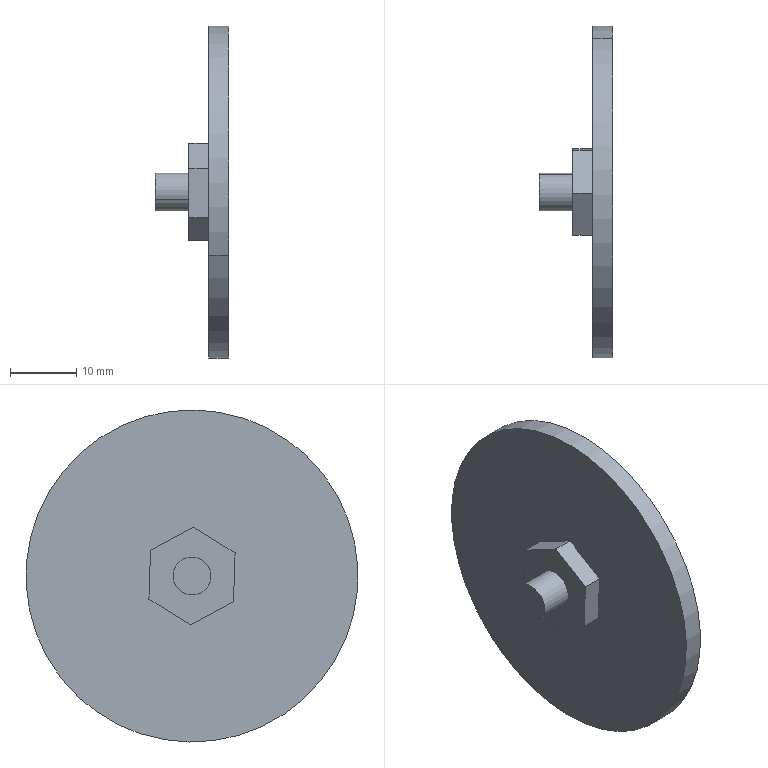Component | SolidWorks | RetainingRing,Gasket,Bolt-4 | 1 solid | 14 faces | box 11 x 50 x 50 mm | volume 6440 mm3 | plane 10 | cylinder 4 | commonest cylinder face diameters 5.711 x2 50 x2
STEP:
#1=CARTESIAN_POINT('',(3.485,0.7067,-4.288));
#2=VERTEX_POINT('',#1);
#3=CARTESIAN_POINT('',(3.485,0.4989,-4.374));
#4=VERTEX_POINT('',#3);
#5=CARTESIAN_POINT('',(3.485,0.6028,-4.331));
#6=DIRECTION('',(-1.,0.,0.));
#7=DIRECTION('',(0.,0.9242,0.3818));
#8=AXIS2_PLACEMENT_3D('',#5,#6,#7);
#9=CIRCLE('',#8,0.1124);
#10=EDGE_CURVE('',#2,#4,#9,.T.);
#11=ORIENTED_EDGE('',*,*,#10,.F.);
#12=CARTESIAN_POINT('',(3.682,0.7067,-4.288));
#13=VERTEX_POINT('',#12);
#14=CARTESIAN_POINT('',(3.485,0.7067,-4.288));
#15=DIRECTION('',(1.,0.,0.));
#16=VECTOR('',#15,39.37);
#17=LINE('',#14,#16);
#18=EDGE_CURVE('',#2,#13,#17,.T.);
#19=ORIENTED_EDGE('',*,*,#18,.T.);
#20=CARTESIAN_POINT('',(3.682,0.4989,-4.374));
#21=VERTEX_POINT('',#20);
#22=CARTESIAN_POINT('',(3.682,0.6028,-4.331));
#23=DIRECTION('',(-1.,0.,0.));
#24=DIRECTION('',(0.,0.9242,0.3818));
#25=AXIS2_PLACEMENT_3D('',#22,#23,#24);
#26=CIRCLE('',#25,0.1124);
#27=EDGE_CURVE('',#13,#21,#26,.T.);
#28=ORIENTED_EDGE('',*,*,#27,.T.);
#29=CARTESIAN_POINT('',(3.485,0.4989,-4.374));
#30=DIRECTION('',(1.,0.,0.));
#31=VECTOR('',#30,39.37);
#32=LINE('',#29,#31);
#33=EDGE_CURVE('',#4,#21,#32,.T.);
#34=ORIENTED_EDGE('',*,*,#33,.F.);
#35=EDGE_LOOP('',(#11,#19,#28,#34));
#36=FACE_OUTER_BOUND('',#35,.T.);
#37=CARTESIAN_POINT('',(3.485,0.6028,-4.331));
#38=DIRECTION('',(1.,0.,0.));
#39=DIRECTION('',(0.,-0.9242,-0.3818));
#40=AXIS2_PLACEMENT_3D('',#37,#38,#39);
#41=CYLINDRICAL_SURFACE('',#40,0.1124);
#42=ADVANCED_FACE('',(#36),#41,.T.);
#43=CARTESIAN_POINT('',(3.8,1.512,-3.955));
#44=VERTEX_POINT('',#43);
#45=CARTESIAN_POINT('',(3.8,-0.3069,-4.707));
#46=VERTEX_POINT('',#45);
#47=CARTESIAN_POINT('',(3.8,0.6028,-4.331));
#48=DIRECTION('',(-1.,0.,0.));
#49=DIRECTION('',(0.,0.9242,0.3818));
#50=AXIS2_PLACEMENT_3D('',#47,#48,#49);
#51=CIRCLE('',#50,0.9843);
#52=EDGE_CURVE('',#44,#46,#51,.T.);
#53=ORIENTED_EDGE('',*,*,#52,.F.);
#54=CARTESIAN_POINT('',(3.918,1.512,-3.955));
#55=VERTEX_POINT('',#54);
#56=CARTESIAN_POINT('',(3.8,1.512,-3.955));
#57=DIRECTION('',(1.,0.,0.));
#58=VECTOR('',#57,39.37);
#59=LINE('',#56,#58);
#60=EDGE_CURVE('',#44,#55,#59,.T.);
#61=ORIENTED_EDGE('',*,*,#60,.T.);
#62=CARTESIAN_POINT('',(3.918,-0.3069,-4.707));
#63=VERTEX_POINT('',#62);
#64=CARTESIAN_POINT('',(3.918,0.6028,-4.331));
#65=DIRECTION('',(-1.,0.,0.));
#66=DIRECTION('',(0.,0.9242,0.3818));
#67=AXIS2_PLACEMENT_3D('',#64,#65,#66);
#68=CIRCLE('',#67,0.9843);
#69=EDGE_CURVE('',#55,#63,#68,.T.);
#70=ORIENTED_EDGE('',*,*,#69,.T.);
#71=CARTESIAN_POINT('',(3.8,-0.3069,-4.707));
#72=DIRECTION('',(1.,0.,0.));
#73=VECTOR('',#72,39.37);
#74=LINE('',#71,#73);
#75=EDGE_CURVE('',#46,#63,#74,.T.);
#76=ORIENTED_EDGE('',*,*,#75,.F.);
#77=EDGE_LOOP('',(#53,#61,#70,#76));
#78=FACE_OUTER_BOUND('',#77,.T.);
#79=CARTESIAN_POINT('',(3.8,0.6028,-4.331));
#80=DIRECTION('',(1.,0.,0.));
#81=DIRECTION('',(0.,-0.9242,-0.3818));
#82=AXIS2_PLACEMENT_3D('',#79,#80,#81);
#83=CYLINDRICAL_SURFACE('',#82,0.9843);
#84=ADVANCED_FACE('',(#78),#83,.T.);
#85=CARTESIAN_POINT('',(3.682,0.3567,-4.483));
#86=VERTEX_POINT('',#85);
#87=CARTESIAN_POINT('',(3.682,0.3474,-4.194));
#88=VERTEX_POINT('',#87);
#89=CARTESIAN_POINT('',(3.682,0.3567,-4.483));
#90=DIRECTION('',(0.,-0.03186,0.9995));
#91=VECTOR('',#90,39.37);
#92=LINE('',#89,#91);
#93=EDGE_CURVE('',#86,#88,#92,.T.);
#94=ORIENTED_EDGE('',*,*,#93,.T.);
#95=CARTESIAN_POINT('',(3.682,0.5935,-4.041));
#96=VERTEX_POINT('',#95);
#97=CARTESIAN_POINT('',(3.682,0.3474,-4.194));
#98=DIRECTION('',(0.,0.8497,0.5273));
#99=VECTOR('',#98,39.37);
#100=LINE('',#97,#99);
#101=EDGE_CURVE('',#88,#96,#100,.T.);
#102=ORIENTED_EDGE('',*,*,#101,.T.);
#103=CARTESIAN_POINT('',(3.682,0.8489,-4.178));
#104=VERTEX_POINT('',#103);
#105=CARTESIAN_POINT('',(3.682,0.5935,-4.041));
#106=DIRECTION('',(0.,0.8815,-0.4722));
#107=VECTOR('',#106,39.37);
#108=LINE('',#105,#107);
#109=EDGE_CURVE('',#96,#104,#108,.T.);
#110=ORIENTED_EDGE('',*,*,#109,.T.);
#111=CARTESIAN_POINT('',(3.682,0.8581,-4.467));
#112=VERTEX_POINT('',#111);
#113=CARTESIAN_POINT('',(3.682,0.8489,-4.178));
#114=DIRECTION('',(0.,0.03186,-0.9995));
#115=VECTOR('',#114,39.37);
#116=LINE('',#113,#115);
#117=EDGE_CURVE('',#104,#112,#116,.T.);
#118=ORIENTED_EDGE('',*,*,#117,.T.);
#119=CARTESIAN_POINT('',(3.682,0.612,-4.62));
#120=VERTEX_POINT('',#119);
#121=CARTESIAN_POINT('',(3.682,0.8581,-4.467));
#122=DIRECTION('',(0.,-0.8497,-0.5273));
#123=VECTOR('',#122,39.37);
#124=LINE('',#121,#123);
#125=EDGE_CURVE('',#112,#120,#124,.T.);
#126=ORIENTED_EDGE('',*,*,#125,.T.);
#127=CARTESIAN_POINT('',(3.682,0.612,-4.62));
#128=DIRECTION('',(0.,-0.8815,0.4722));
#129=VECTOR('',#128,39.37);
#130=LINE('',#127,#129);
#131=EDGE_CURVE('',#120,#86,#130,.T.);
#132=ORIENTED_EDGE('',*,*,#131,.T.);
#133=EDGE_LOOP('',(#94,#102,#110,#118,#126,#132));
#134=FACE_OUTER_BOUND('',#133,.T.);
#135=CARTESIAN_POINT('',(3.682,0.6028,-4.331));
#136=DIRECTION('',(-1.,0.,0.));
#137=DIRECTION('',(0.,0.9242,0.3818));
#138=AXIS2_PLACEMENT_3D('',#135,#136,#137);
#139=CIRCLE('',#138,0.1124);
#140=EDGE_CURVE('',#21,#13,#139,.T.);
#141=ORIENTED_EDGE('',*,*,#140,.F.);
#142=ORIENTED_EDGE('',*,*,#27,.F.);
#143=EDGE_LOOP('',(#141,#142));
#144=FACE_BOUND('',#143,.T.);
#145=CARTESIAN_POINT('',(3.682,0.6028,-4.331));
#146=DIRECTION('',(-1.,0.,0.));
#147=DIRECTION('',(0.,0.9242,0.3818));
#148=AXIS2_PLACEMENT_3D('',#145,#146,#147);
#149=PLANE('',#148);
#150=ADVANCED_FACE('',(#134,#144),#149,.T.);
#151=CARTESIAN_POINT('',(3.8,0.6028,-4.331));
#152=DIRECTION('',(-1.,0.,0.));
#153=DIRECTION('',(0.,0.9242,0.3818));
#154=AXIS2_PLACEMENT_3D('',#151,#152,#153);
#155=CIRCLE('',#154,0.9843);
#156=EDGE_CURVE('',#46,#44,#155,.T.);
#157=ORIENTED_EDGE('',*,*,#156,.T.);
#158=ORIENTED_EDGE('',*,*,#52,.T.);
#159=EDGE_LOOP('',(#157,#158));
#160=FACE_OUTER_BOUND('',#159,.T.);
#161=CARTESIAN_POINT('',(3.8,0.3474,-4.194));
#162=VERTEX_POINT('',#161);
#163=CARTESIAN_POINT('',(3.8,0.5935,-4.041));
#164=VERTEX_POINT('',#163);
#165=CARTESIAN_POINT('',(3.8,0.3474,-4.194));
#166=DIRECTION('',(0.,0.8497,0.5273));
#167=VECTOR('',#166,39.37);
#168=LINE('',#165,#167);
#169=EDGE_CURVE('',#162,#164,#168,.T.);
#170=ORIENTED_EDGE('',*,*,#169,.F.);
#171=CARTESIAN_POINT('',(3.8,0.3567,-4.483));
#172=VERTEX_POINT('',#171);
#173=CARTESIAN_POINT('',(3.8,0.3567,-4.483));
#174=DIRECTION('',(0.,-0.03186,0.9995));
#175=VECTOR('',#174,39.37);
#176=LINE('',#173,#175);
#177=EDGE_CURVE('',#172,#162,#176,.T.);
#178=ORIENTED_EDGE('',*,*,#177,.F.);
#179=CARTESIAN_POINT('',(3.8,0.612,-4.62));
#180=VERTEX_POINT('',#179);
#181=CARTESIAN_POINT('',(3.8,0.612,-4.62));
#182=DIRECTION('',(0.,-0.8815,0.4722));
#183=VECTOR('',#182,39.37);
#184=LINE('',#181,#183);
#185=EDGE_CURVE('',#180,#172,#184,.T.);
#186=ORIENTED_EDGE('',*,*,#185,.F.);
#187=CARTESIAN_POINT('',(3.8,0.8581,-4.467));
#188=VERTEX_POINT('',#187);
#189=CARTESIAN_POINT('',(3.8,0.8581,-4.467));
#190=DIRECTION('',(0.,-0.8497,-0.5273));
#191=VECTOR('',#190,39.37);
#192=LINE('',#189,#191);
#193=EDGE_CURVE('',#188,#180,#192,.T.);
#194=ORIENTED_EDGE('',*,*,#193,.F.);
#195=CARTESIAN_POINT('',(3.8,0.8489,-4.178));
#196=VERTEX_POINT('',#195);
#197=CARTESIAN_POINT('',(3.8,0.8489,-4.178));
#198=DIRECTION('',(0.,0.03186,-0.9995));
#199=VECTOR('',#198,39.37);
#200=LINE('',#197,#199);
#201=EDGE_CURVE('',#196,#188,#200,.T.);
#202=ORIENTED_EDGE('',*,*,#201,.F.);
#203=CARTESIAN_POINT('',(3.8,0.5935,-4.041));
#204=DIRECTION('',(0.,0.8815,-0.4722));
#205=VECTOR('',#204,39.37);
#206=LINE('',#203,#205);
#207=EDGE_CURVE('',#164,#196,#206,.T.);
#208=ORIENTED_EDGE('',*,*,#207,.F.);
#209=EDGE_LOOP('',(#170,#178,#186,#194,#202,#208));
#210=FACE_BOUND('',#209,.T.);
#211=CARTESIAN_POINT('',(3.8,0.6028,-4.331));
#212=DIRECTION('',(-1.,0.,0.));
#213=DIRECTION('',(0.,0.9242,0.3818));
#214=AXIS2_PLACEMENT_3D('',#211,#212,#213);
#215=PLANE('',#214);
#216=ADVANCED_FACE('',(#160,#210),#215,.T.);
#217=ORIENTED_EDGE('',*,*,#60,.F.);
#218=ORIENTED_EDGE('',*,*,#156,.F.);
#219=ORIENTED_EDGE('',*,*,#75,.T.);
#220=CARTESIAN_POINT('',(3.918,0.6028,-4.331));
#221=DIRECTION('',(-1.,0.,0.));
#222=DIRECTION('',(0.,0.9242,0.3818));
#223=AXIS2_PLACEMENT_3D('',#220,#221,#222);
#224=CIRCLE('',#223,0.9843);
#225=EDGE_CURVE('',#63,#55,#224,.T.);
#226=ORIENTED_EDGE('',*,*,#225,.T.);
#227=EDGE_LOOP('',(#217,#218,#219,#226));
#228=FACE_OUTER_BOUND('',#227,.T.);
#229=CARTESIAN_POINT('',(3.8,0.6028,-4.331));
#230=DIRECTION('',(1.,0.,0.));
#231=DIRECTION('',(0.,-0.9242,-0.3818));
#232=AXIS2_PLACEMENT_3D('',#229,#230,#231);
#233=CYLINDRICAL_SURFACE('',#232,0.9843);
#234=ADVANCED_FACE('',(#228),#233,.T.);
#235=ORIENTED_EDGE('',*,*,#225,.F.);
#236=ORIENTED_EDGE('',*,*,#69,.F.);
#237=EDGE_LOOP('',(#235,#236));
#238=FACE_OUTER_BOUND('',#237,.T.);
#239=CARTESIAN_POINT('',(3.918,0.6028,-4.331));
#240=DIRECTION('',(-1.,0.,0.));
#241=DIRECTION('',(0.,0.9242,0.3818));
#242=AXIS2_PLACEMENT_3D('',#239,#240,#241);
#243=PLANE('',#242);
#244=ADVANCED_FACE('',(#238),#243,.F.);
#245=ORIENTED_EDGE('',*,*,#177,.T.);
#246=CARTESIAN_POINT('',(3.682,0.3474,-4.194));
#247=DIRECTION('',(1.,0.,0.));
#248=VECTOR('',#247,39.37);
#249=LINE('',#246,#248);
#250=EDGE_CURVE('',#88,#162,#249,.T.);
#251=ORIENTED_EDGE('',*,*,#250,.F.);
#252=ORIENTED_EDGE('',*,*,#93,.F.);
#253=CARTESIAN_POINT('',(3.682,0.3567,-4.483));
#254=DIRECTION('',(1.,0.,0.));
#255=VECTOR('',#254,39.37);
#256=LINE('',#253,#255);
#257=EDGE_CURVE('',#86,#172,#256,.T.);
#258=ORIENTED_EDGE('',*,*,#257,.T.);
#259=EDGE_LOOP('',(#245,#251,#252,#258));
#260=FACE_OUTER_BOUND('',#259,.T.);
#261=CARTESIAN_POINT('',(3.682,0.3567,-4.483));
#262=DIRECTION('',(0.,0.9995,0.03186));
#263=DIRECTION('',(0.,0.03186,-0.9995));
#264=AXIS2_PLACEMENT_3D('',#261,#262,#263);
#265=PLANE('',#264);
#266=ADVANCED_FACE('',(#260),#265,.F.);
#267=ORIENTED_EDGE('',*,*,#169,.T.);
#268=CARTESIAN_POINT('',(3.682,0.5935,-4.041));
#269=DIRECTION('',(1.,0.,0.));
#270=VECTOR('',#269,39.37);
#271=LINE('',#268,#270);
#272=EDGE_CURVE('',#96,#164,#271,.T.);
#273=ORIENTED_EDGE('',*,*,#272,.F.);
#274=ORIENTED_EDGE('',*,*,#101,.F.);
#275=ORIENTED_EDGE('',*,*,#250,.T.);
#276=EDGE_LOOP('',(#267,#273,#274,#275));
#277=FACE_OUTER_BOUND('',#276,.T.);
#278=CARTESIAN_POINT('',(3.682,0.3474,-4.194));
#279=DIRECTION('',(0.,0.5273,-0.8497));
#280=DIRECTION('',(0.,-0.8497,-0.5273));
#281=AXIS2_PLACEMENT_3D('',#278,#279,#280);
#282=PLANE('',#281);
#283=ADVANCED_FACE('',(#277),#282,.F.);
#284=ORIENTED_EDGE('',*,*,#207,.T.);
#285=CARTESIAN_POINT('',(3.682,0.8489,-4.178));
#286=DIRECTION('',(1.,0.,0.));
#287=VECTOR('',#286,39.37);
#288=LINE('',#285,#287);
#289=EDGE_CURVE('',#104,#196,#288,.T.);
#290=ORIENTED_EDGE('',*,*,#289,.F.);
#291=ORIENTED_EDGE('',*,*,#109,.F.);
#292=ORIENTED_EDGE('',*,*,#272,.T.);
#293=EDGE_LOOP('',(#284,#290,#291,#292));
#294=FACE_OUTER_BOUND('',#293,.T.);
#295=CARTESIAN_POINT('',(3.682,0.5935,-4.041));
#296=DIRECTION('',(0.,-0.4722,-0.8815));
#297=DIRECTION('',(0.,-0.8815,0.4722));
#298=AXIS2_PLACEMENT_3D('',#295,#296,#297);
#299=PLANE('',#298);
#300=ADVANCED_FACE('',(#294),#299,.F.);
#301=ORIENTED_EDGE('',*,*,#201,.T.);
#302=CARTESIAN_POINT('',(3.682,0.8581,-4.467));
#303=DIRECTION('',(1.,0.,0.));
#304=VECTOR('',#303,39.37);
#305=LINE('',#302,#304);
#306=EDGE_CURVE('',#112,#188,#305,.T.);
#307=ORIENTED_EDGE('',*,*,#306,.F.);
#308=ORIENTED_EDGE('',*,*,#117,.F.);
#309=ORIENTED_EDGE('',*,*,#289,.T.);
#310=EDGE_LOOP('',(#301,#307,#308,#309));
#311=FACE_OUTER_BOUND('',#310,.T.);
#312=CARTESIAN_POINT('',(3.682,0.8489,-4.178));
#313=DIRECTION('',(0.,-0.9995,-0.03186));
#314=DIRECTION('',(0.,-0.03186,0.9995));
#315=AXIS2_PLACEMENT_3D('',#312,#313,#314);
#316=PLANE('',#315);
#317=ADVANCED_FACE('',(#311),#316,.F.);
#318=ORIENTED_EDGE('',*,*,#193,.T.);
#319=CARTESIAN_POINT('',(3.682,0.612,-4.62));
#320=DIRECTION('',(1.,0.,0.));
#321=VECTOR('',#320,39.37);
#322=LINE('',#319,#321);
#323=EDGE_CURVE('',#120,#180,#322,.T.);
#324=ORIENTED_EDGE('',*,*,#323,.F.);
#325=ORIENTED_EDGE('',*,*,#125,.F.);
#326=ORIENTED_EDGE('',*,*,#306,.T.);
#327=EDGE_LOOP('',(#318,#324,#325,#326));
#328=FACE_OUTER_BOUND('',#327,.T.);
#329=CARTESIAN_POINT('',(3.682,0.8581,-4.467));
#330=DIRECTION('',(0.,-0.5273,0.8497));
#331=DIRECTION('',(0.,0.8497,0.5273));
#332=AXIS2_PLACEMENT_3D('',#329,#330,#331);
#333=PLANE('',#332);
#334=ADVANCED_FACE('',(#328),#333,.F.);
#335=ORIENTED_EDGE('',*,*,#185,.T.);
#336=ORIENTED_EDGE('',*,*,#257,.F.);
#337=ORIENTED_EDGE('',*,*,#131,.F.);
#338=ORIENTED_EDGE('',*,*,#323,.T.);
#339=EDGE_LOOP('',(#335,#336,#337,#338));
#340=FACE_OUTER_BOUND('',#339,.T.);
#341=CARTESIAN_POINT('',(3.682,0.612,-4.62));
#342=DIRECTION('',(0.,0.4722,0.8815));
#343=DIRECTION('',(0.,0.8815,-0.4722));
#344=AXIS2_PLACEMENT_3D('',#341,#342,#343);
#345=PLANE('',#344);
#346=ADVANCED_FACE('',(#340),#345,.F.);
#347=ORIENTED_EDGE('',*,*,#18,.F.);
#348=CARTESIAN_POINT('',(3.485,0.6028,-4.331));
#349=DIRECTION('',(-1.,0.,0.));
#350=DIRECTION('',(0.,0.9242,0.3818));
#351=AXIS2_PLACEMENT_3D('',#348,#349,#350);
#352=CIRCLE('',#351,0.1124);
#353=EDGE_CURVE('',#4,#2,#352,.T.);
#354=ORIENTED_EDGE('',*,*,#353,.F.);
#355=ORIENTED_EDGE('',*,*,#33,.T.);
#356=ORIENTED_EDGE('',*,*,#140,.T.);
#357=EDGE_LOOP('',(#347,#354,#355,#356));
#358=FACE_OUTER_BOUND('',#357,.T.);
#359=CARTESIAN_POINT('',(3.485,0.6028,-4.331));
#360=DIRECTION('',(1.,0.,0.));
#361=DIRECTION('',(0.,-0.9242,-0.3818));
#362=AXIS2_PLACEMENT_3D('',#359,#360,#361);
#363=CYLINDRICAL_SURFACE('',#362,0.1124);
#364=ADVANCED_FACE('',(#358),#363,.T.);
#365=ORIENTED_EDGE('',*,*,#353,.T.);
#366=ORIENTED_EDGE('',*,*,#10,.T.);
#367=EDGE_LOOP('',(#365,#366));
#368=FACE_OUTER_BOUND('',#367,.T.);
#369=CARTESIAN_POINT('',(3.485,0.6028,-4.331));
#370=DIRECTION('',(-1.,0.,0.));
#371=DIRECTION('',(0.,0.9242,0.3818));
#372=AXIS2_PLACEMENT_3D('',#369,#370,#371);
#373=PLANE('',#372);
#374=ADVANCED_FACE('',(#368),#373,.T.);
#375=CLOSED_SHELL('',(#42,#84,#150,#216,#234,#244,#266,#283,#300,#317,#334,#346,#364,#374));
#376=MANIFOLD_SOLID_BREP('',#375);
#377=CARTESIAN_POINT('',(0.,0.,0.));
#378=DIRECTION('',(0.,0.,1.));
#379=DIRECTION('',(1.,0.,0.));
#380=AXIS2_PLACEMENT_3D('',#377,#378,#379);
#381=(LENGTH_UNIT()NAMED_UNIT(*)SI_UNIT($,.METRE.));
#382=LENGTH_MEASURE_WITH_UNIT(LENGTH_MEASURE(0.0254),#381);
#383=DIMENSIONAL_EXPONENTS(1.,0.,0.,0.,0.,0.,0.);
#384=(CONVERSION_BASED_UNIT('',#382)LENGTH_UNIT()NAMED_UNIT(#383));
#385=UNCERTAINTY_MEASURE_WITH_UNIT(LENGTH_MEASURE(0.00001),#384,'','');
#386=(NAMED_UNIT(*)PLANE_ANGLE_UNIT()SI_UNIT($,.RADIAN.));
#387=(NAMED_UNIT(*)SI_UNIT($,.STERADIAN.)SOLID_ANGLE_UNIT());
#388=(GEOMETRIC_REPRESENTATION_CONTEXT(3)GLOBAL_UNCERTAINTY_ASSIGNED_CONTEXT((#385))GLOBAL_UNIT_ASSIGNED_CONTEXT((#384,#386,#387))REPRESENTATION_CONTEXT('',''));
#389=ADVANCED_BREP_SHAPE_REPRESENTATION('',(#376,#380),#388);
#390=COLOUR_RGB('',0.7922,0.8196,0.9333);
#391=FILL_AREA_STYLE_COLOUR('',#390);
#392=FILL_AREA_STYLE('',(#391));
#393=SURFACE_STYLE_FILL_AREA(#392);
#394=SURFACE_SIDE_STYLE('',(#393));
#395=SURFACE_STYLE_USAGE(.BOTH.,#394);
#396=PRESENTATION_STYLE_ASSIGNMENT((#395));
#397=STYLED_ITEM('',(#396),#376);
#398=(LENGTH_UNIT()NAMED_UNIT(*)SI_UNIT($,.METRE.));
#399=LENGTH_MEASURE_WITH_UNIT(LENGTH_MEASURE(0.0254),#398);
#400=DIMENSIONAL_EXPONENTS(1.,0.,0.,0.,0.,0.,0.);
#401=(CONVERSION_BASED_UNIT('',#399)LENGTH_UNIT()NAMED_UNIT(#400));
#402=UNCERTAINTY_MEASURE_WITH_UNIT(LENGTH_MEASURE(0.00001),#401,'','');
#403=(NAMED_UNIT(*)PLANE_ANGLE_UNIT()SI_UNIT($,.RADIAN.));
#404=(NAMED_UNIT(*)SI_UNIT($,.STERADIAN.)SOLID_ANGLE_UNIT());
#405=(GEOMETRIC_REPRESENTATION_CONTEXT(3)GLOBAL_UNCERTAINTY_ASSIGNED_CONTEXT((#402))GLOBAL_UNIT_ASSIGNED_CONTEXT((#401,#403,#404))REPRESENTATION_CONTEXT('',''));
#406=MECHANICAL_DESIGN_GEOMETRIC_PRESENTATION_REPRESENTATION('',(#397),#405);
#407=PRESENTATION_LAYER_ASSIGNMENT('','',(#397));